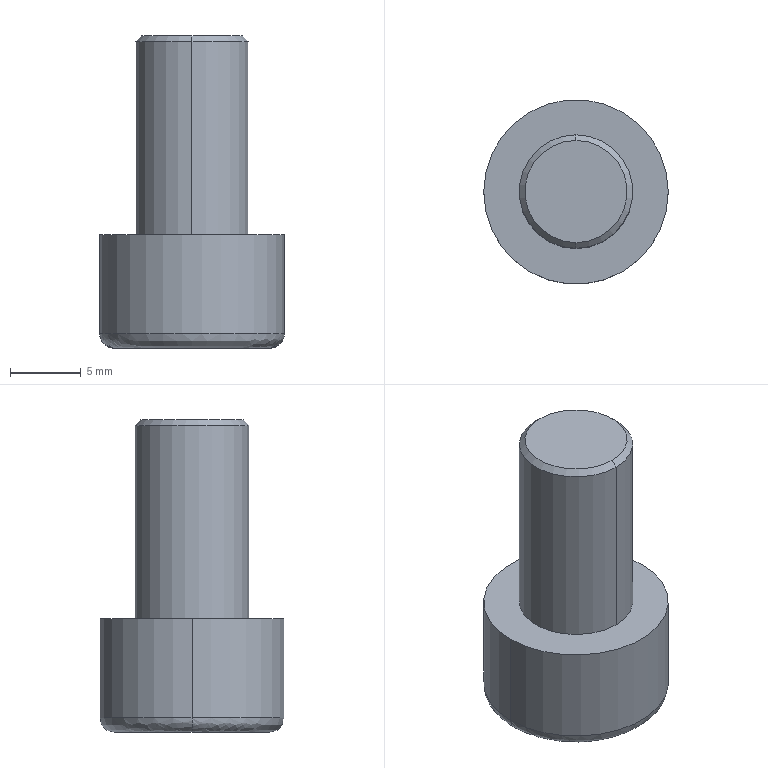Component | SolidWorks | M8x14HexSocket-1 | 1 solid | 25 faces | box 13 x 13 x 22 mm | volume 1614 mm3 | plane 15 | cone 4 | cylinder 4 | spline 2 | commonest cylinder face diameters 8 x2 13 x2
STEP:
#1=CARTESIAN_POINT('',(-19.808,-4.877,92.457));
#2=VERTEX_POINT('',#1);
#3=CARTESIAN_POINT('',(-19.296,-4.877,92.457));
#4=VERTEX_POINT('',#3);
#5=CARTESIAN_POINT('',(-19.552,-4.877,92.457));
#6=DIRECTION('',(0.,0.,1.));
#7=DIRECTION('',(-1.,0.,0.));
#8=AXIS2_PLACEMENT_3D('',#5,#6,#7);
#9=CIRCLE('',#8,0.2559);
#10=EDGE_CURVE('',#2,#4,#9,.T.);
#11=ORIENTED_EDGE('',*,*,#10,.F.);
#12=CARTESIAN_POINT('',(-19.768,-4.877,92.417));
#13=VERTEX_POINT('',#12);
#14=CARTESIAN_POINT('',(-19.768,-4.877,92.457));
#15=DIRECTION('',(-0.,-1.,0.));
#16=DIRECTION('',(-1.,0.,0.));
#17=AXIS2_PLACEMENT_3D('',#14,#15,#16);
#18=CIRCLE('',#17,0.03937);
#19=EDGE_CURVE('',#2,#13,#18,.T.);
#20=ORIENTED_EDGE('',*,*,#19,.T.);
#21=CARTESIAN_POINT('',(-19.335,-4.877,92.417));
#22=VERTEX_POINT('',#21);
#23=CARTESIAN_POINT('',(-19.768,-4.877,92.417));
#24=CARTESIAN_POINT('',(-19.768,-5.31,92.417));
#25=CARTESIAN_POINT('',(-19.335,-5.31,92.417));
#26=CARTESIAN_POINT('',(-19.335,-4.877,92.417));
#27=(BOUNDED_CURVE()B_SPLINE_CURVE(3,(#23,#24,#25,#26),.UNSPECIFIED.,.F.,.F.)B_SPLINE_CURVE_WITH_KNOTS((4,4),(0.,1.),.UNSPECIFIED.)CURVE()GEOMETRIC_REPRESENTATION_ITEM()RATIONAL_B_SPLINE_CURVE((1.,0.3333,0.3333,1.))REPRESENTATION_ITEM(''));
#28=EDGE_CURVE('',#13,#22,#27,.T.);
#29=ORIENTED_EDGE('',*,*,#28,.T.);
#30=CARTESIAN_POINT('',(-19.335,-4.877,92.457));
#31=DIRECTION('',(0.,1.,-0.));
#32=DIRECTION('',(1.,0.,0.));
#33=AXIS2_PLACEMENT_3D('',#30,#31,#32);
#34=CIRCLE('',#33,0.03937);
#35=EDGE_CURVE('',#4,#22,#34,.T.);
#36=ORIENTED_EDGE('',*,*,#35,.F.);
#37=EDGE_LOOP('',(#11,#20,#29,#36));
#38=FACE_OUTER_BOUND('',#37,.T.);
#39=CARTESIAN_POINT('',(-19.808,-4.877,92.457));
#40=CARTESIAN_POINT('',(-19.808,-5.389,92.457));
#41=CARTESIAN_POINT('',(-19.296,-5.389,92.457));
#42=CARTESIAN_POINT('',(-19.296,-4.877,92.457));
#43=CARTESIAN_POINT('',(-19.808,-4.877,92.434));
#44=CARTESIAN_POINT('',(-19.808,-5.389,92.434));
#45=CARTESIAN_POINT('',(-19.296,-5.389,92.434));
#46=CARTESIAN_POINT('',(-19.296,-4.877,92.434));
#47=CARTESIAN_POINT('',(-19.791,-4.877,92.417));
#48=CARTESIAN_POINT('',(-19.791,-5.356,92.417));
#49=CARTESIAN_POINT('',(-19.312,-5.356,92.417));
#50=CARTESIAN_POINT('',(-19.312,-4.877,92.417));
#51=CARTESIAN_POINT('',(-19.768,-4.877,92.417));
#52=CARTESIAN_POINT('',(-19.768,-5.31,92.417));
#53=CARTESIAN_POINT('',(-19.335,-5.31,92.417));
#54=CARTESIAN_POINT('',(-19.335,-4.877,92.417));
#55=(BOUNDED_SURFACE()B_SPLINE_SURFACE(3,3,((#39,#40,#41,#42),(#43,#44,#45,#46),(#47,#48,#49,#50),(#51,#52,#53,#54)),.UNSPECIFIED.,.F.,.F.,.F.)B_SPLINE_SURFACE_WITH_KNOTS((4,4),(4,4),(0.,1.),(0.,1.),.UNSPECIFIED.)GEOMETRIC_REPRESENTATION_ITEM()RATIONAL_B_SPLINE_SURFACE(((1.,0.3333,0.3333,1.),(0.8047,0.2682,0.2682,0.8047),(0.8047,0.2682,0.2682,0.8047),(1.,0.3333,0.3333,1.)))REPRESENTATION_ITEM('')SURFACE());
#56=ADVANCED_FACE('',(#38),#55,.T.);
#57=CARTESIAN_POINT('',(-19.552,-4.735,93.283));
#58=VERTEX_POINT('',#57);
#59=CARTESIAN_POINT('',(-19.552,-5.019,93.283));
#60=VERTEX_POINT('',#59);
#61=CARTESIAN_POINT('',(-19.552,-4.877,93.283));
#62=DIRECTION('',(0.,-0.,1.));
#63=DIRECTION('',(0.,1.,0.));
#64=AXIS2_PLACEMENT_3D('',#61,#62,#63);
#65=CIRCLE('',#64,0.1417);
#66=EDGE_CURVE('',#58,#60,#65,.T.);
#67=ORIENTED_EDGE('',*,*,#66,.F.);
#68=CARTESIAN_POINT('',(-19.552,-4.719,93.268));
#69=VERTEX_POINT('',#68);
#70=CARTESIAN_POINT('',(-19.552,-4.719,93.268));
#71=DIRECTION('',(0.,0.7071,-0.7071));
#72=VECTOR('',#71,39.37);
#73=LINE('',#70,#72);
#74=EDGE_CURVE('',#58,#69,#73,.T.);
#75=ORIENTED_EDGE('',*,*,#74,.T.);
#76=CARTESIAN_POINT('',(-19.552,-5.034,93.268));
#77=VERTEX_POINT('',#76);
#78=CARTESIAN_POINT('',(-19.552,-4.877,93.268));
#79=DIRECTION('',(-0.,0.,-1.));
#80=DIRECTION('',(0.,1.,0.));
#81=AXIS2_PLACEMENT_3D('',#78,#79,#80);
#82=CIRCLE('',#81,0.1575);
#83=EDGE_CURVE('',#77,#69,#82,.T.);
#84=ORIENTED_EDGE('',*,*,#83,.F.);
#85=CARTESIAN_POINT('',(-19.552,-5.034,93.268));
#86=DIRECTION('',(-0.,-0.7071,-0.7071));
#87=VECTOR('',#86,39.37);
#88=LINE('',#85,#87);
#89=EDGE_CURVE('',#60,#77,#88,.T.);
#90=ORIENTED_EDGE('',*,*,#89,.F.);
#91=EDGE_LOOP('',(#67,#75,#84,#90));
#92=FACE_OUTER_BOUND('',#91,.T.);
#93=CARTESIAN_POINT('',(-19.552,-4.877,93.268));
#94=DIRECTION('',(-0.,0.,-1.));
#95=DIRECTION('',(0.,-1.,0.));
#96=AXIS2_PLACEMENT_3D('',#93,#94,#95);
#97=CONICAL_SURFACE('',#96,0.1575,0.7854);
#98=ADVANCED_FACE('',(#92),#97,.T.);
#99=ORIENTED_EDGE('',*,*,#83,.T.);
#100=CARTESIAN_POINT('',(-19.552,-4.719,92.732));
#101=VERTEX_POINT('',#100);
#102=CARTESIAN_POINT('',(-19.552,-4.719,93.283));
#103=DIRECTION('',(0.,0.,-1.));
#104=VECTOR('',#103,39.37);
#105=LINE('',#102,#104);
#106=EDGE_CURVE('',#69,#101,#105,.T.);
#107=ORIENTED_EDGE('',*,*,#106,.T.);
#108=CARTESIAN_POINT('',(-19.552,-5.034,92.732));
#109=VERTEX_POINT('',#108);
#110=CARTESIAN_POINT('',(-19.552,-4.877,92.732));
#111=DIRECTION('',(0.,0.,1.));
#112=DIRECTION('',(1.,0.,0.));
#113=AXIS2_PLACEMENT_3D('',#110,#111,#112);
#114=CIRCLE('',#113,0.1575);
#115=EDGE_CURVE('',#101,#109,#114,.T.);
#116=ORIENTED_EDGE('',*,*,#115,.T.);
#117=CARTESIAN_POINT('',(-19.552,-5.034,93.283));
#118=DIRECTION('',(0.,0.,-1.));
#119=VECTOR('',#118,39.37);
#120=LINE('',#117,#119);
#121=EDGE_CURVE('',#77,#109,#120,.T.);
#122=ORIENTED_EDGE('',*,*,#121,.F.);
#123=EDGE_LOOP('',(#99,#107,#116,#122));
#124=FACE_OUTER_BOUND('',#123,.T.);
#125=CARTESIAN_POINT('',(-19.552,-4.877,93.283));
#126=DIRECTION('',(0.,0.,-1.));
#127=DIRECTION('',(0.,-1.,0.));
#128=AXIS2_PLACEMENT_3D('',#125,#126,#127);
#129=CYLINDRICAL_SURFACE('',#128,0.1575);
#130=ADVANCED_FACE('',(#124),#129,.T.);
#131=CARTESIAN_POINT('',(-19.296,-4.877,92.732));
#132=VERTEX_POINT('',#131);
#133=CARTESIAN_POINT('',(-19.808,-4.877,92.732));
#134=VERTEX_POINT('',#133);
#135=CARTESIAN_POINT('',(-19.552,-4.877,92.732));
#136=DIRECTION('',(0.,0.,1.));
#137=DIRECTION('',(-1.,0.,0.));
#138=AXIS2_PLACEMENT_3D('',#135,#136,#137);
#139=CIRCLE('',#138,0.2559);
#140=EDGE_CURVE('',#132,#134,#139,.T.);
#141=ORIENTED_EDGE('',*,*,#140,.F.);
#142=CARTESIAN_POINT('',(-19.296,-4.877,92.732));
#143=DIRECTION('',(-0.,-0.,-1.));
#144=VECTOR('',#143,39.37);
#145=LINE('',#142,#144);
#146=EDGE_CURVE('',#132,#4,#145,.T.);
#147=ORIENTED_EDGE('',*,*,#146,.T.);
#148=CARTESIAN_POINT('',(-19.552,-4.877,92.457));
#149=DIRECTION('',(0.,0.,1.));
#150=DIRECTION('',(-1.,0.,0.));
#151=AXIS2_PLACEMENT_3D('',#148,#149,#150);
#152=CIRCLE('',#151,0.2559);
#153=EDGE_CURVE('',#4,#2,#152,.T.);
#154=ORIENTED_EDGE('',*,*,#153,.T.);
#155=CARTESIAN_POINT('',(-19.808,-4.877,92.732));
#156=DIRECTION('',(-0.,-0.,-1.));
#157=VECTOR('',#156,39.37);
#158=LINE('',#155,#157);
#159=EDGE_CURVE('',#134,#2,#158,.T.);
#160=ORIENTED_EDGE('',*,*,#159,.F.);
#161=EDGE_LOOP('',(#141,#147,#154,#160));
#162=FACE_OUTER_BOUND('',#161,.T.);
#163=CARTESIAN_POINT('',(-19.552,-4.877,92.732));
#164=DIRECTION('',(-0.,-0.,-1.));
#165=DIRECTION('',(-1.,0.,0.));
#166=AXIS2_PLACEMENT_3D('',#163,#164,#165);
#167=CYLINDRICAL_SURFACE('',#166,0.2559);
#168=ADVANCED_FACE('',(#162),#167,.T.);
#169=CARTESIAN_POINT('',(-19.552,-4.877,92.643));
#170=VERTEX_POINT('',#169);
#171=CARTESIAN_POINT('',(-19.67,-4.877,92.575));
#172=VERTEX_POINT('',#171);
#173=CARTESIAN_POINT('',(-19.67,-4.877,92.575));
#174=DIRECTION('',(-0.866,0.,-0.5));
#175=VECTOR('',#174,39.37);
#176=LINE('',#173,#175);
#177=EDGE_CURVE('',#170,#172,#176,.T.);
#178=ORIENTED_EDGE('',*,*,#177,.F.);
#179=CARTESIAN_POINT('',(-19.434,-4.877,92.575));
#180=VERTEX_POINT('',#179);
#181=CARTESIAN_POINT('',(-19.434,-4.877,92.575));
#182=DIRECTION('',(0.866,-0.,-0.5));
#183=VECTOR('',#182,39.37);
#184=LINE('',#181,#183);
#185=EDGE_CURVE('',#170,#180,#184,.T.);
#186=ORIENTED_EDGE('',*,*,#185,.T.);
#187=CARTESIAN_POINT('',(-19.449,-4.936,92.575));
#188=VERTEX_POINT('',#187);
#189=CARTESIAN_POINT('',(-19.552,-4.877,92.575));
#190=DIRECTION('',(0.,0.,1.));
#191=DIRECTION('',(-1.,0.,0.));
#192=AXIS2_PLACEMENT_3D('',#189,#190,#191);
#193=CIRCLE('',#192,0.1181);
#194=EDGE_CURVE('',#188,#180,#193,.T.);
#195=ORIENTED_EDGE('',*,*,#194,.F.);
#196=CARTESIAN_POINT('',(-19.552,-4.995,92.575));
#197=VERTEX_POINT('',#196);
#198=CARTESIAN_POINT('',(-19.552,-4.877,92.575));
#199=DIRECTION('',(0.,0.,1.));
#200=DIRECTION('',(-1.,-0.,0.));
#201=AXIS2_PLACEMENT_3D('',#198,#199,#200);
#202=CIRCLE('',#201,0.1181);
#203=EDGE_CURVE('',#197,#188,#202,.T.);
#204=ORIENTED_EDGE('',*,*,#203,.F.);
#205=CARTESIAN_POINT('',(-19.654,-4.936,92.575));
#206=VERTEX_POINT('',#205);
#207=CARTESIAN_POINT('',(-19.552,-4.877,92.575));
#208=DIRECTION('',(-0.,-0.,-1.));
#209=DIRECTION('',(-1.,0.,0.));
#210=AXIS2_PLACEMENT_3D('',#207,#208,#209);
#211=CIRCLE('',#210,0.1181);
#212=EDGE_CURVE('',#197,#206,#211,.T.);
#213=ORIENTED_EDGE('',*,*,#212,.T.);
#214=CARTESIAN_POINT('',(-19.552,-4.877,92.575));
#215=DIRECTION('',(0.,0.,1.));
#216=DIRECTION('',(-1.,0.,0.));
#217=AXIS2_PLACEMENT_3D('',#214,#215,#216);
#218=CIRCLE('',#217,0.1181);
#219=EDGE_CURVE('',#172,#206,#218,.T.);
#220=ORIENTED_EDGE('',*,*,#219,.F.);
#221=EDGE_LOOP('',(#178,#186,#195,#204,#213,#220));
#222=FACE_OUTER_BOUND('',#221,.T.);
#223=CARTESIAN_POINT('',(-19.552,-4.877,92.575));
#224=DIRECTION('',(-0.,-0.,-1.));
#225=DIRECTION('',(-1.,0.,0.));
#226=AXIS2_PLACEMENT_3D('',#223,#224,#225);
#227=CONICAL_SURFACE('',#226,0.1181,1.047);
#228=ADVANCED_FACE('',(#222),#227,.F.);
#229=CARTESIAN_POINT('',(-19.552,-4.877,92.732));
#230=DIRECTION('',(0.,0.,1.));
#231=DIRECTION('',(1.,0.,0.));
#232=AXIS2_PLACEMENT_3D('',#229,#230,#231);
#233=CIRCLE('',#232,0.1575);
#234=EDGE_CURVE('',#109,#101,#233,.T.);
#235=ORIENTED_EDGE('',*,*,#234,.F.);
#236=ORIENTED_EDGE('',*,*,#115,.F.);
#237=EDGE_LOOP('',(#235,#236));
#238=FACE_BOUND('',#237,.T.);
#239=CARTESIAN_POINT('',(-19.552,-4.877,92.732));
#240=DIRECTION('',(0.,0.,1.));
#241=DIRECTION('',(-1.,0.,0.));
#242=AXIS2_PLACEMENT_3D('',#239,#240,#241);
#243=CIRCLE('',#242,0.2559);
#244=EDGE_CURVE('',#134,#132,#243,.T.);
#245=ORIENTED_EDGE('',*,*,#244,.T.);
#246=ORIENTED_EDGE('',*,*,#140,.T.);
#247=EDGE_LOOP('',(#245,#246));
#248=FACE_OUTER_BOUND('',#247,.T.);
#249=CARTESIAN_POINT('',(-19.552,-4.877,92.732));
#250=DIRECTION('',(0.,0.,1.));
#251=DIRECTION('',(1.,-0.,-0.));
#252=AXIS2_PLACEMENT_3D('',#249,#250,#251);
#253=PLANE('',#252);
#254=ADVANCED_FACE('',(#238,#248),#253,.T.);
#255=ORIENTED_EDGE('',*,*,#146,.F.);
#256=ORIENTED_EDGE('',*,*,#244,.F.);
#257=ORIENTED_EDGE('',*,*,#159,.T.);
#258=ORIENTED_EDGE('',*,*,#10,.T.);
#259=EDGE_LOOP('',(#255,#256,#257,#258));
#260=FACE_OUTER_BOUND('',#259,.T.);
#261=CARTESIAN_POINT('',(-19.552,-4.877,92.732));
#262=DIRECTION('',(-0.,-0.,-1.));
#263=DIRECTION('',(-1.,0.,0.));
#264=AXIS2_PLACEMENT_3D('',#261,#262,#263);
#265=CYLINDRICAL_SURFACE('',#264,0.2559);
#266=ADVANCED_FACE('',(#260),#265,.T.);
#267=ORIENTED_EDGE('',*,*,#19,.F.);
#268=ORIENTED_EDGE('',*,*,#153,.F.);
#269=ORIENTED_EDGE('',*,*,#35,.T.);
#270=CARTESIAN_POINT('',(-19.335,-4.877,92.417));
#271=CARTESIAN_POINT('',(-19.335,-4.444,92.417));
#272=CARTESIAN_POINT('',(-19.768,-4.444,92.417));
#273=CARTESIAN_POINT('',(-19.768,-4.877,92.417));
#274=(BOUNDED_CURVE()B_SPLINE_CURVE(3,(#270,#271,#272,#273),.UNSPECIFIED.,.F.,.F.)B_SPLINE_CURVE_WITH_KNOTS((4,4),(0.,1.),.UNSPECIFIED.)CURVE()GEOMETRIC_REPRESENTATION_ITEM()RATIONAL_B_SPLINE_CURVE((1.,0.3333,0.3333,1.))REPRESENTATION_ITEM(''));
#275=EDGE_CURVE('',#22,#13,#274,.T.);
#276=ORIENTED_EDGE('',*,*,#275,.T.);
#277=EDGE_LOOP('',(#267,#268,#269,#276));
#278=FACE_OUTER_BOUND('',#277,.T.);
#279=CARTESIAN_POINT('',(-19.296,-4.877,92.457));
#280=CARTESIAN_POINT('',(-19.296,-4.365,92.457));
#281=CARTESIAN_POINT('',(-19.808,-4.365,92.457));
#282=CARTESIAN_POINT('',(-19.808,-4.877,92.457));
#283=CARTESIAN_POINT('',(-19.296,-4.877,92.434));
#284=CARTESIAN_POINT('',(-19.296,-4.365,92.434));
#285=CARTESIAN_POINT('',(-19.808,-4.365,92.434));
#286=CARTESIAN_POINT('',(-19.808,-4.877,92.434));
#287=CARTESIAN_POINT('',(-19.312,-4.877,92.417));
#288=CARTESIAN_POINT('',(-19.312,-4.398,92.417));
#289=CARTESIAN_POINT('',(-19.791,-4.398,92.417));
#290=CARTESIAN_POINT('',(-19.791,-4.877,92.417));
#291=CARTESIAN_POINT('',(-19.335,-4.877,92.417));
#292=CARTESIAN_POINT('',(-19.335,-4.444,92.417));
#293=CARTESIAN_POINT('',(-19.768,-4.444,92.417));
#294=CARTESIAN_POINT('',(-19.768,-4.877,92.417));
#295=(BOUNDED_SURFACE()B_SPLINE_SURFACE(3,3,((#279,#280,#281,#282),(#283,#284,#285,#286),(#287,#288,#289,#290),(#291,#292,#293,#294)),.UNSPECIFIED.,.F.,.F.,.F.)B_SPLINE_SURFACE_WITH_KNOTS((4,4),(4,4),(0.,1.),(0.,1.),.UNSPECIFIED.)GEOMETRIC_REPRESENTATION_ITEM()RATIONAL_B_SPLINE_SURFACE(((1.,0.3333,0.3333,1.),(0.8047,0.2682,0.2682,0.8047),(0.8047,0.2682,0.2682,0.8047),(1.,0.3333,0.3333,1.)))REPRESENTATION_ITEM('')SURFACE());
#296=ADVANCED_FACE('',(#278),#295,.T.);
#297=CARTESIAN_POINT('',(-19.483,-4.759,92.417));
#298=VERTEX_POINT('',#297);
#299=CARTESIAN_POINT('',(-19.415,-4.877,92.417));
#300=VERTEX_POINT('',#299);
#301=CARTESIAN_POINT('',(-19.483,-4.759,92.417));
#302=DIRECTION('',(0.5,-0.866,0.));
#303=VECTOR('',#302,39.37);
#304=LINE('',#301,#303);
#305=EDGE_CURVE('',#298,#300,#304,.T.);
#306=ORIENTED_EDGE('',*,*,#305,.F.);
#307=CARTESIAN_POINT('',(-19.62,-4.759,92.417));
#308=VERTEX_POINT('',#307);
#309=CARTESIAN_POINT('',(-19.552,-4.759,92.417));
#310=DIRECTION('',(1.,-0.,-0.));
#311=VECTOR('',#310,39.37);
#312=LINE('',#309,#311);
#313=EDGE_CURVE('',#308,#298,#312,.T.);
#314=ORIENTED_EDGE('',*,*,#313,.F.);
#315=CARTESIAN_POINT('',(-19.688,-4.877,92.417));
#316=VERTEX_POINT('',#315);
#317=CARTESIAN_POINT('',(-19.688,-4.877,92.417));
#318=DIRECTION('',(0.5,0.866,-0.));
#319=VECTOR('',#318,39.37);
#320=LINE('',#317,#319);
#321=EDGE_CURVE('',#316,#308,#320,.T.);
#322=ORIENTED_EDGE('',*,*,#321,.F.);
#323=CARTESIAN_POINT('',(-19.62,-4.995,92.417));
#324=VERTEX_POINT('',#323);
#325=CARTESIAN_POINT('',(-19.62,-4.995,92.417));
#326=DIRECTION('',(-0.5,0.866,-0.));
#327=VECTOR('',#326,39.37);
#328=LINE('',#325,#327);
#329=EDGE_CURVE('',#324,#316,#328,.T.);
#330=ORIENTED_EDGE('',*,*,#329,.F.);
#331=CARTESIAN_POINT('',(-19.483,-4.995,92.417));
#332=VERTEX_POINT('',#331);
#333=CARTESIAN_POINT('',(-19.552,-4.995,92.417));
#334=DIRECTION('',(-1.,0.,0.));
#335=VECTOR('',#334,39.37);
#336=LINE('',#333,#335);
#337=EDGE_CURVE('',#332,#324,#336,.T.);
#338=ORIENTED_EDGE('',*,*,#337,.F.);
#339=CARTESIAN_POINT('',(-19.415,-4.877,92.417));
#340=DIRECTION('',(-0.5,-0.866,0.));
#341=VECTOR('',#340,39.37);
#342=LINE('',#339,#341);
#343=EDGE_CURVE('',#300,#332,#342,.T.);
#344=ORIENTED_EDGE('',*,*,#343,.F.);
#345=EDGE_LOOP('',(#306,#314,#322,#330,#338,#344));
#346=FACE_BOUND('',#345,.T.);
#347=ORIENTED_EDGE('',*,*,#275,.F.);
#348=ORIENTED_EDGE('',*,*,#28,.F.);
#349=EDGE_LOOP('',(#347,#348));
#350=FACE_OUTER_BOUND('',#349,.T.);
#351=CARTESIAN_POINT('',(-19.552,-4.877,92.417));
#352=DIRECTION('',(0.,0.,1.));
#353=DIRECTION('',(1.,-0.,-0.));
#354=AXIS2_PLACEMENT_3D('',#351,#352,#353);
#355=PLANE('',#354);
#356=ADVANCED_FACE('',(#346,#350),#355,.F.);
#357=CARTESIAN_POINT('',(-19.415,-4.877,92.575));
#358=VERTEX_POINT('',#357);
#359=CARTESIAN_POINT('',(-19.483,-4.995,92.575));
#360=DIRECTION('',(0.5,0.866,-0.));
#361=VECTOR('',#360,39.37);
#362=LINE('',#359,#361);
#363=EDGE_CURVE('',#188,#358,#362,.T.);
#364=ORIENTED_EDGE('',*,*,#363,.T.);
#365=CARTESIAN_POINT('',(-19.415,-4.877,92.575));
#366=DIRECTION('',(-0.,-0.,-1.));
#367=VECTOR('',#366,39.37);
#368=LINE('',#365,#367);
#369=EDGE_CURVE('',#358,#300,#368,.T.);
#370=ORIENTED_EDGE('',*,*,#369,.T.);
#371=ORIENTED_EDGE('',*,*,#343,.T.);
#372=CARTESIAN_POINT('',(-19.483,-4.995,92.575));
#373=VERTEX_POINT('',#372);
#374=CARTESIAN_POINT('',(-19.483,-4.995,92.575));
#375=DIRECTION('',(0.,0.,1.));
#376=VECTOR('',#375,39.37);
#377=LINE('',#374,#376);
#378=EDGE_CURVE('',#332,#373,#377,.T.);
#379=ORIENTED_EDGE('',*,*,#378,.T.);
#380=CARTESIAN_POINT('',(-19.483,-4.995,92.575));
#381=DIRECTION('',(0.5,0.866,-0.));
#382=VECTOR('',#381,39.37);
#383=LINE('',#380,#382);
#384=EDGE_CURVE('',#373,#188,#383,.T.);
#385=ORIENTED_EDGE('',*,*,#384,.T.);
#386=EDGE_LOOP('',(#364,#370,#371,#379,#385));
#387=FACE_OUTER_BOUND('',#386,.T.);
#388=CARTESIAN_POINT('',(-19.483,-4.995,92.575));
#389=DIRECTION('',(-0.866,0.5,-0.));
#390=DIRECTION('',(-0.5,-0.866,0.));
#391=AXIS2_PLACEMENT_3D('',#388,#389,#390);
#392=PLANE('',#391);
#393=ADVANCED_FACE('',(#387),#392,.T.);
#394=CARTESIAN_POINT('',(-19.449,-4.818,92.575));
#395=VERTEX_POINT('',#394);
#396=CARTESIAN_POINT('',(-19.483,-4.759,92.575));
#397=VERTEX_POINT('',#396);
#398=CARTESIAN_POINT('',(-19.449,-4.818,92.575));
#399=DIRECTION('',(-0.5,0.866,-0.));
#400=VECTOR('',#399,39.37);
#401=LINE('',#398,#400);
#402=EDGE_CURVE('',#395,#397,#401,.T.);
#403=ORIENTED_EDGE('',*,*,#402,.T.);
#404=CARTESIAN_POINT('',(-19.483,-4.759,92.575));
#405=DIRECTION('',(-0.,-0.,-1.));
#406=VECTOR('',#405,39.37);
#407=LINE('',#404,#406);
#408=EDGE_CURVE('',#397,#298,#407,.T.);
#409=ORIENTED_EDGE('',*,*,#408,.T.);
#410=ORIENTED_EDGE('',*,*,#305,.T.);
#411=ORIENTED_EDGE('',*,*,#369,.F.);
#412=CARTESIAN_POINT('',(-19.415,-4.877,92.575));
#413=DIRECTION('',(-0.5,0.866,-0.));
#414=VECTOR('',#413,39.37);
#415=LINE('',#412,#414);
#416=EDGE_CURVE('',#358,#395,#415,.T.);
#417=ORIENTED_EDGE('',*,*,#416,.T.);
#418=EDGE_LOOP('',(#403,#409,#410,#411,#417));
#419=FACE_OUTER_BOUND('',#418,.T.);
#420=CARTESIAN_POINT('',(-19.415,-4.877,92.575));
#421=DIRECTION('',(-0.866,-0.5,0.));
#422=DIRECTION('',(0.5,-0.866,0.));
#423=AXIS2_PLACEMENT_3D('',#420,#421,#422);
#424=PLANE('',#423);
#425=ADVANCED_FACE('',(#419),#424,.T.);
#426=CARTESIAN_POINT('',(-19.552,-4.759,92.575));
#427=VERTEX_POINT('',#426);
#428=CARTESIAN_POINT('',(-19.62,-4.759,92.575));
#429=VERTEX_POINT('',#428);
#430=CARTESIAN_POINT('',(-19.415,-4.759,92.575));
#431=DIRECTION('',(-1.,0.,0.));
#432=VECTOR('',#431,39.37);
#433=LINE('',#430,#432);
#434=EDGE_CURVE('',#427,#429,#433,.T.);
#435=ORIENTED_EDGE('',*,*,#434,.T.);
#436=CARTESIAN_POINT('',(-19.62,-4.759,92.575));
#437=DIRECTION('',(-0.,-0.,-1.));
#438=VECTOR('',#437,39.37);
#439=LINE('',#436,#438);
#440=EDGE_CURVE('',#429,#308,#439,.T.);
#441=ORIENTED_EDGE('',*,*,#440,.T.);
#442=ORIENTED_EDGE('',*,*,#313,.T.);
#443=ORIENTED_EDGE('',*,*,#408,.F.);
#444=CARTESIAN_POINT('',(-19.415,-4.759,92.575));
#445=DIRECTION('',(-1.,0.,0.));
#446=VECTOR('',#445,39.37);
#447=LINE('',#444,#446);
#448=EDGE_CURVE('',#397,#427,#447,.T.);
#449=ORIENTED_EDGE('',*,*,#448,.T.);
#450=EDGE_LOOP('',(#435,#441,#442,#443,#449));
#451=FACE_OUTER_BOUND('',#450,.T.);
#452=CARTESIAN_POINT('',(-19.483,-4.759,92.575));
#453=DIRECTION('',(-0.,-1.,0.));
#454=DIRECTION('',(1.,-0.,-0.));
#455=AXIS2_PLACEMENT_3D('',#452,#453,#454);
#456=PLANE('',#455);
#457=ADVANCED_FACE('',(#451),#456,.T.);
#458=CARTESIAN_POINT('',(-19.654,-4.818,92.575));
#459=VERTEX_POINT('',#458);
#460=CARTESIAN_POINT('',(-19.688,-4.877,92.575));
#461=VERTEX_POINT('',#460);
#462=CARTESIAN_POINT('',(-19.62,-4.759,92.575));
#463=DIRECTION('',(-0.5,-0.866,0.));
#464=VECTOR('',#463,39.37);
#465=LINE('',#462,#464);
#466=EDGE_CURVE('',#459,#461,#465,.T.);
#467=ORIENTED_EDGE('',*,*,#466,.T.);
#468=CARTESIAN_POINT('',(-19.688,-4.877,92.575));
#469=DIRECTION('',(-0.,-0.,-1.));
#470=VECTOR('',#469,39.37);
#471=LINE('',#468,#470);
#472=EDGE_CURVE('',#461,#316,#471,.T.);
#473=ORIENTED_EDGE('',*,*,#472,.T.);
#474=ORIENTED_EDGE('',*,*,#321,.T.);
#475=ORIENTED_EDGE('',*,*,#440,.F.);
#476=CARTESIAN_POINT('',(-19.62,-4.759,92.575));
#477=DIRECTION('',(-0.5,-0.866,0.));
#478=VECTOR('',#477,39.37);
#479=LINE('',#476,#478);
#480=EDGE_CURVE('',#429,#459,#479,.T.);
#481=ORIENTED_EDGE('',*,*,#480,.T.);
#482=EDGE_LOOP('',(#467,#473,#474,#475,#481));
#483=FACE_OUTER_BOUND('',#482,.T.);
#484=CARTESIAN_POINT('',(-19.62,-4.759,92.575));
#485=DIRECTION('',(0.866,-0.5,0.));
#486=DIRECTION('',(0.5,0.866,-0.));
#487=AXIS2_PLACEMENT_3D('',#484,#485,#486);
#488=PLANE('',#487);
#489=ADVANCED_FACE('',(#483),#488,.T.);
#490=CARTESIAN_POINT('',(-19.62,-4.995,92.575));
#491=VERTEX_POINT('',#490);
#492=CARTESIAN_POINT('',(-19.688,-4.877,92.575));
#493=DIRECTION('',(0.5,-0.866,0.));
#494=VECTOR('',#493,39.37);
#495=LINE('',#492,#494);
#496=EDGE_CURVE('',#206,#491,#495,.T.);
#497=ORIENTED_EDGE('',*,*,#496,.T.);
#498=CARTESIAN_POINT('',(-19.62,-4.995,92.575));
#499=DIRECTION('',(-0.,-0.,-1.));
#500=VECTOR('',#499,39.37);
#501=LINE('',#498,#500);
#502=EDGE_CURVE('',#491,#324,#501,.T.);
#503=ORIENTED_EDGE('',*,*,#502,.T.);
#504=ORIENTED_EDGE('',*,*,#329,.T.);
#505=ORIENTED_EDGE('',*,*,#472,.F.);
#506=CARTESIAN_POINT('',(-19.688,-4.877,92.575));
#507=DIRECTION('',(0.5,-0.866,0.));
#508=VECTOR('',#507,39.37);
#509=LINE('',#506,#508);
#510=EDGE_CURVE('',#461,#206,#509,.T.);
#511=ORIENTED_EDGE('',*,*,#510,.T.);
#512=EDGE_LOOP('',(#497,#503,#504,#505,#511));
#513=FACE_OUTER_BOUND('',#512,.T.);
#514=CARTESIAN_POINT('',(-19.688,-4.877,92.575));
#515=DIRECTION('',(0.866,0.5,-0.));
#516=DIRECTION('',(-0.5,0.866,-0.));
#517=AXIS2_PLACEMENT_3D('',#514,#515,#516);
#518=PLANE('',#517);
#519=ADVANCED_FACE('',(#513),#518,.T.);
#520=CARTESIAN_POINT('',(-19.415,-4.995,92.575));
#521=DIRECTION('',(1.,-0.,-0.));
#522=VECTOR('',#521,39.37);
#523=LINE('',#520,#522);
#524=EDGE_CURVE('',#197,#373,#523,.T.);
#525=ORIENTED_EDGE('',*,*,#524,.T.);
#526=ORIENTED_EDGE('',*,*,#378,.F.);
#527=ORIENTED_EDGE('',*,*,#337,.T.);
#528=ORIENTED_EDGE('',*,*,#502,.F.);
#529=CARTESIAN_POINT('',(-19.62,-4.995,92.575));
#530=DIRECTION('',(1.,-0.,0.));
#531=VECTOR('',#530,39.37);
#532=LINE('',#529,#531);
#533=EDGE_CURVE('',#491,#197,#532,.T.);
#534=ORIENTED_EDGE('',*,*,#533,.T.);
#535=EDGE_LOOP('',(#525,#526,#527,#528,#534));
#536=FACE_OUTER_BOUND('',#535,.T.);
#537=CARTESIAN_POINT('',(-19.62,-4.995,92.575));
#538=DIRECTION('',(0.,1.,-0.));
#539=DIRECTION('',(-1.,0.,-0.));
#540=AXIS2_PLACEMENT_3D('',#537,#538,#539);
#541=PLANE('',#540);
#542=ADVANCED_FACE('',(#536),#541,.T.);
#543=ORIENTED_EDGE('',*,*,#416,.F.);
#544=ORIENTED_EDGE('',*,*,#363,.F.);
#545=ORIENTED_EDGE('',*,*,#194,.T.);
#546=CARTESIAN_POINT('',(-19.552,-4.877,92.575));
#547=DIRECTION('',(0.,0.,1.));
#548=DIRECTION('',(-1.,0.,0.));
#549=AXIS2_PLACEMENT_3D('',#546,#547,#548);
#550=CIRCLE('',#549,0.1181);
#551=EDGE_CURVE('',#180,#395,#550,.T.);
#552=ORIENTED_EDGE('',*,*,#551,.T.);
#553=EDGE_LOOP('',(#543,#544,#545,#552));
#554=FACE_OUTER_BOUND('',#553,.T.);
#555=CARTESIAN_POINT('',(-19.415,-4.877,92.575));
#556=DIRECTION('',(0.,0.,1.));
#557=DIRECTION('',(1.,-0.,-0.));
#558=AXIS2_PLACEMENT_3D('',#555,#556,#557);
#559=PLANE('',#558);
#560=ADVANCED_FACE('',(#554),#559,.F.);
#561=ORIENTED_EDGE('',*,*,#510,.F.);
#562=ORIENTED_EDGE('',*,*,#466,.F.);
#563=CARTESIAN_POINT('',(-19.552,-4.877,92.575));
#564=DIRECTION('',(0.,0.,1.));
#565=DIRECTION('',(-1.,0.,0.));
#566=AXIS2_PLACEMENT_3D('',#563,#564,#565);
#567=CIRCLE('',#566,0.1181);
#568=EDGE_CURVE('',#459,#172,#567,.T.);
#569=ORIENTED_EDGE('',*,*,#568,.T.);
#570=ORIENTED_EDGE('',*,*,#219,.T.);
#571=EDGE_LOOP('',(#561,#562,#569,#570));
#572=FACE_OUTER_BOUND('',#571,.T.);
#573=CARTESIAN_POINT('',(-19.415,-4.877,92.575));
#574=DIRECTION('',(0.,0.,1.));
#575=DIRECTION('',(1.,-0.,-0.));
#576=AXIS2_PLACEMENT_3D('',#573,#574,#575);
#577=PLANE('',#576);
#578=ADVANCED_FACE('',(#572),#577,.F.);
#579=ORIENTED_EDGE('',*,*,#533,.F.);
#580=ORIENTED_EDGE('',*,*,#496,.F.);
#581=ORIENTED_EDGE('',*,*,#212,.F.);
#582=EDGE_LOOP('',(#579,#580,#581));
#583=FACE_OUTER_BOUND('',#582,.T.);
#584=CARTESIAN_POINT('',(-19.415,-4.877,92.575));
#585=DIRECTION('',(0.,0.,1.));
#586=DIRECTION('',(1.,-0.,-0.));
#587=AXIS2_PLACEMENT_3D('',#584,#585,#586);
#588=PLANE('',#587);
#589=ADVANCED_FACE('',(#583),#588,.F.);
#590=ORIENTED_EDGE('',*,*,#185,.F.);
#591=ORIENTED_EDGE('',*,*,#177,.T.);
#592=ORIENTED_EDGE('',*,*,#568,.F.);
#593=CARTESIAN_POINT('',(-19.552,-4.877,92.575));
#594=DIRECTION('',(0.,0.,1.));
#595=DIRECTION('',(-1.,-0.,0.));
#596=AXIS2_PLACEMENT_3D('',#593,#594,#595);
#597=CIRCLE('',#596,0.1181);
#598=EDGE_CURVE('',#427,#459,#597,.T.);
#599=ORIENTED_EDGE('',*,*,#598,.F.);
#600=CARTESIAN_POINT('',(-19.552,-4.877,92.575));
#601=DIRECTION('',(0.,0.,1.));
#602=DIRECTION('',(-1.,-0.,0.));
#603=AXIS2_PLACEMENT_3D('',#600,#601,#602);
#604=CIRCLE('',#603,0.1181);
#605=EDGE_CURVE('',#395,#427,#604,.T.);
#606=ORIENTED_EDGE('',*,*,#605,.F.);
#607=ORIENTED_EDGE('',*,*,#551,.F.);
#608=EDGE_LOOP('',(#590,#591,#592,#599,#606,#607));
#609=FACE_OUTER_BOUND('',#608,.T.);
#610=CARTESIAN_POINT('',(-19.552,-4.877,92.575));
#611=DIRECTION('',(-0.,-0.,-1.));
#612=DIRECTION('',(-1.,0.,0.));
#613=AXIS2_PLACEMENT_3D('',#610,#611,#612);
#614=CONICAL_SURFACE('',#613,0.1181,1.047);
#615=ADVANCED_FACE('',(#609),#614,.F.);
#616=ORIENTED_EDGE('',*,*,#384,.F.);
#617=ORIENTED_EDGE('',*,*,#524,.F.);
#618=ORIENTED_EDGE('',*,*,#203,.T.);
#619=EDGE_LOOP('',(#616,#617,#618));
#620=FACE_OUTER_BOUND('',#619,.T.);
#621=CARTESIAN_POINT('',(-19.415,-4.877,92.575));
#622=DIRECTION('',(0.,0.,1.));
#623=DIRECTION('',(1.,-0.,-0.));
#624=AXIS2_PLACEMENT_3D('',#621,#622,#623);
#625=PLANE('',#624);
#626=ADVANCED_FACE('',(#620),#625,.F.);
#627=ORIENTED_EDGE('',*,*,#480,.F.);
#628=ORIENTED_EDGE('',*,*,#434,.F.);
#629=ORIENTED_EDGE('',*,*,#598,.T.);
#630=EDGE_LOOP('',(#627,#628,#629));
#631=FACE_OUTER_BOUND('',#630,.T.);
#632=CARTESIAN_POINT('',(-19.415,-4.877,92.575));
#633=DIRECTION('',(0.,0.,1.));
#634=DIRECTION('',(1.,-0.,-0.));
#635=AXIS2_PLACEMENT_3D('',#632,#633,#634);
#636=PLANE('',#635);
#637=ADVANCED_FACE('',(#631),#636,.F.);
#638=ORIENTED_EDGE('',*,*,#448,.F.);
#639=ORIENTED_EDGE('',*,*,#402,.F.);
#640=ORIENTED_EDGE('',*,*,#605,.T.);
#641=EDGE_LOOP('',(#638,#639,#640));
#642=FACE_OUTER_BOUND('',#641,.T.);
#643=CARTESIAN_POINT('',(-19.415,-4.877,92.575));
#644=DIRECTION('',(0.,0.,1.));
#645=DIRECTION('',(1.,-0.,-0.));
#646=AXIS2_PLACEMENT_3D('',#643,#644,#645);
#647=PLANE('',#646);
#648=ADVANCED_FACE('',(#642),#647,.F.);
#649=ORIENTED_EDGE('',*,*,#106,.F.);
#650=CARTESIAN_POINT('',(-19.552,-4.877,93.268));
#651=DIRECTION('',(-0.,0.,-1.));
#652=DIRECTION('',(0.,1.,0.));
#653=AXIS2_PLACEMENT_3D('',#650,#651,#652);
#654=CIRCLE('',#653,0.1575);
#655=EDGE_CURVE('',#69,#77,#654,.T.);
#656=ORIENTED_EDGE('',*,*,#655,.T.);
#657=ORIENTED_EDGE('',*,*,#121,.T.);
#658=ORIENTED_EDGE('',*,*,#234,.T.);
#659=EDGE_LOOP('',(#649,#656,#657,#658));
#660=FACE_OUTER_BOUND('',#659,.T.);
#661=CARTESIAN_POINT('',(-19.552,-4.877,93.283));
#662=DIRECTION('',(0.,0.,-1.));
#663=DIRECTION('',(0.,-1.,0.));
#664=AXIS2_PLACEMENT_3D('',#661,#662,#663);
#665=CYLINDRICAL_SURFACE('',#664,0.1575);
#666=ADVANCED_FACE('',(#660),#665,.T.);
#667=CARTESIAN_POINT('',(-19.552,-4.877,93.283));
#668=DIRECTION('',(0.,-0.,1.));
#669=DIRECTION('',(0.,1.,0.));
#670=AXIS2_PLACEMENT_3D('',#667,#668,#669);
#671=CIRCLE('',#670,0.1417);
#672=EDGE_CURVE('',#60,#58,#671,.T.);
#673=ORIENTED_EDGE('',*,*,#672,.T.);
#674=ORIENTED_EDGE('',*,*,#66,.T.);
#675=EDGE_LOOP('',(#673,#674));
#676=FACE_OUTER_BOUND('',#675,.T.);
#677=CARTESIAN_POINT('',(-19.552,-4.719,93.283));
#678=DIRECTION('',(-0.,-0.,1.));
#679=DIRECTION('',(0.,1.,0.));
#680=AXIS2_PLACEMENT_3D('',#677,#678,#679);
#681=PLANE('',#680);
#682=ADVANCED_FACE('',(#676),#681,.T.);
#683=ORIENTED_EDGE('',*,*,#74,.F.);
#684=ORIENTED_EDGE('',*,*,#672,.F.);
#685=ORIENTED_EDGE('',*,*,#89,.T.);
#686=ORIENTED_EDGE('',*,*,#655,.F.);
#687=EDGE_LOOP('',(#683,#684,#685,#686));
#688=FACE_OUTER_BOUND('',#687,.T.);
#689=CARTESIAN_POINT('',(-19.552,-4.877,93.268));
#690=DIRECTION('',(-0.,0.,-1.));
#691=DIRECTION('',(0.,-1.,0.));
#692=AXIS2_PLACEMENT_3D('',#689,#690,#691);
#693=CONICAL_SURFACE('',#692,0.1575,0.7854);
#694=ADVANCED_FACE('',(#688),#693,.T.);
#695=CLOSED_SHELL('',(#56,#98,#130,#168,#228,#254,#266,#296,#356,#393,#425,#457,#489,#519,#542,#560,#578,#589,#615,#626,#637,#648,#666,#682,#694));
#696=MANIFOLD_SOLID_BREP('',#695);
#697=CARTESIAN_POINT('',(0.,0.,0.));
#698=DIRECTION('',(0.,0.,1.));
#699=DIRECTION('',(1.,0.,0.));
#700=AXIS2_PLACEMENT_3D('',#697,#698,#699);
#701=(LENGTH_UNIT()NAMED_UNIT(*)SI_UNIT($,.METRE.));
#702=LENGTH_MEASURE_WITH_UNIT(LENGTH_MEASURE(0.0254),#701);
#703=DIMENSIONAL_EXPONENTS(1.,0.,0.,0.,0.,0.,0.);
#704=(CONVERSION_BASED_UNIT('',#702)LENGTH_UNIT()NAMED_UNIT(#703));
#705=UNCERTAINTY_MEASURE_WITH_UNIT(LENGTH_MEASURE(0.00001),#704,'','');
#706=(NAMED_UNIT(*)PLANE_ANGLE_UNIT()SI_UNIT($,.RADIAN.));
#707=(NAMED_UNIT(*)SI_UNIT($,.STERADIAN.)SOLID_ANGLE_UNIT());
#708=(GEOMETRIC_REPRESENTATION_CONTEXT(3)GLOBAL_UNCERTAINTY_ASSIGNED_CONTEXT((#705))GLOBAL_UNIT_ASSIGNED_CONTEXT((#704,#706,#707))REPRESENTATION_CONTEXT('',''));
#709=ADVANCED_BREP_SHAPE_REPRESENTATION('',(#696,#700),#708);
#710=COLOUR_RGB('',0.7922,0.8196,0.9333);
#711=FILL_AREA_STYLE_COLOUR('',#710);
#712=FILL_AREA_STYLE('',(#711));
#713=SURFACE_STYLE_FILL_AREA(#712);
#714=SURFACE_SIDE_STYLE('',(#713));
#715=SURFACE_STYLE_USAGE(.BOTH.,#714);
#716=PRESENTATION_STYLE_ASSIGNMENT((#715));
#717=STYLED_ITEM('',(#716),#696);
#718=(LENGTH_UNIT()NAMED_UNIT(*)SI_UNIT($,.METRE.));
#719=LENGTH_MEASURE_WITH_UNIT(LENGTH_MEASURE(0.0254),#718);
#720=DIMENSIONAL_EXPONENTS(1.,0.,0.,0.,0.,0.,0.);
#721=(CONVERSION_BASED_UNIT('',#719)LENGTH_UNIT()NAMED_UNIT(#720));
#722=UNCERTAINTY_MEASURE_WITH_UNIT(LENGTH_MEASURE(0.00001),#721,'','');
#723=(NAMED_UNIT(*)PLANE_ANGLE_UNIT()SI_UNIT($,.RADIAN.));
#724=(NAMED_UNIT(*)SI_UNIT($,.STERADIAN.)SOLID_ANGLE_UNIT());
#725=(GEOMETRIC_REPRESENTATION_CONTEXT(3)GLOBAL_UNCERTAINTY_ASSIGNED_CONTEXT((#722))GLOBAL_UNIT_ASSIGNED_CONTEXT((#721,#723,#724))REPRESENTATION_CONTEXT('',''));
#726=MECHANICAL_DESIGN_GEOMETRIC_PRESENTATION_REPRESENTATION('',(#717),#725);
#727=PRESENTATION_LAYER_ASSIGNMENT('','',(#717));